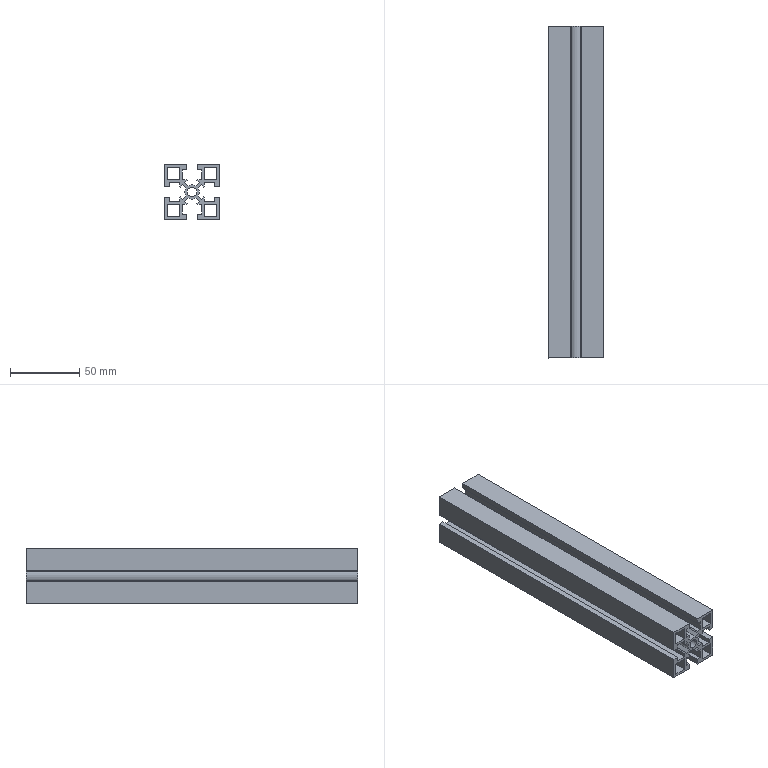Component | SolidWorks | Profile240-4 | 1 solid | 89 faces | volume 139218 mm3 | plane 82 | cylinder 7 | commonest cylinder face diameters 10.5 x5 6.8 x2 | material 6061 Alloy